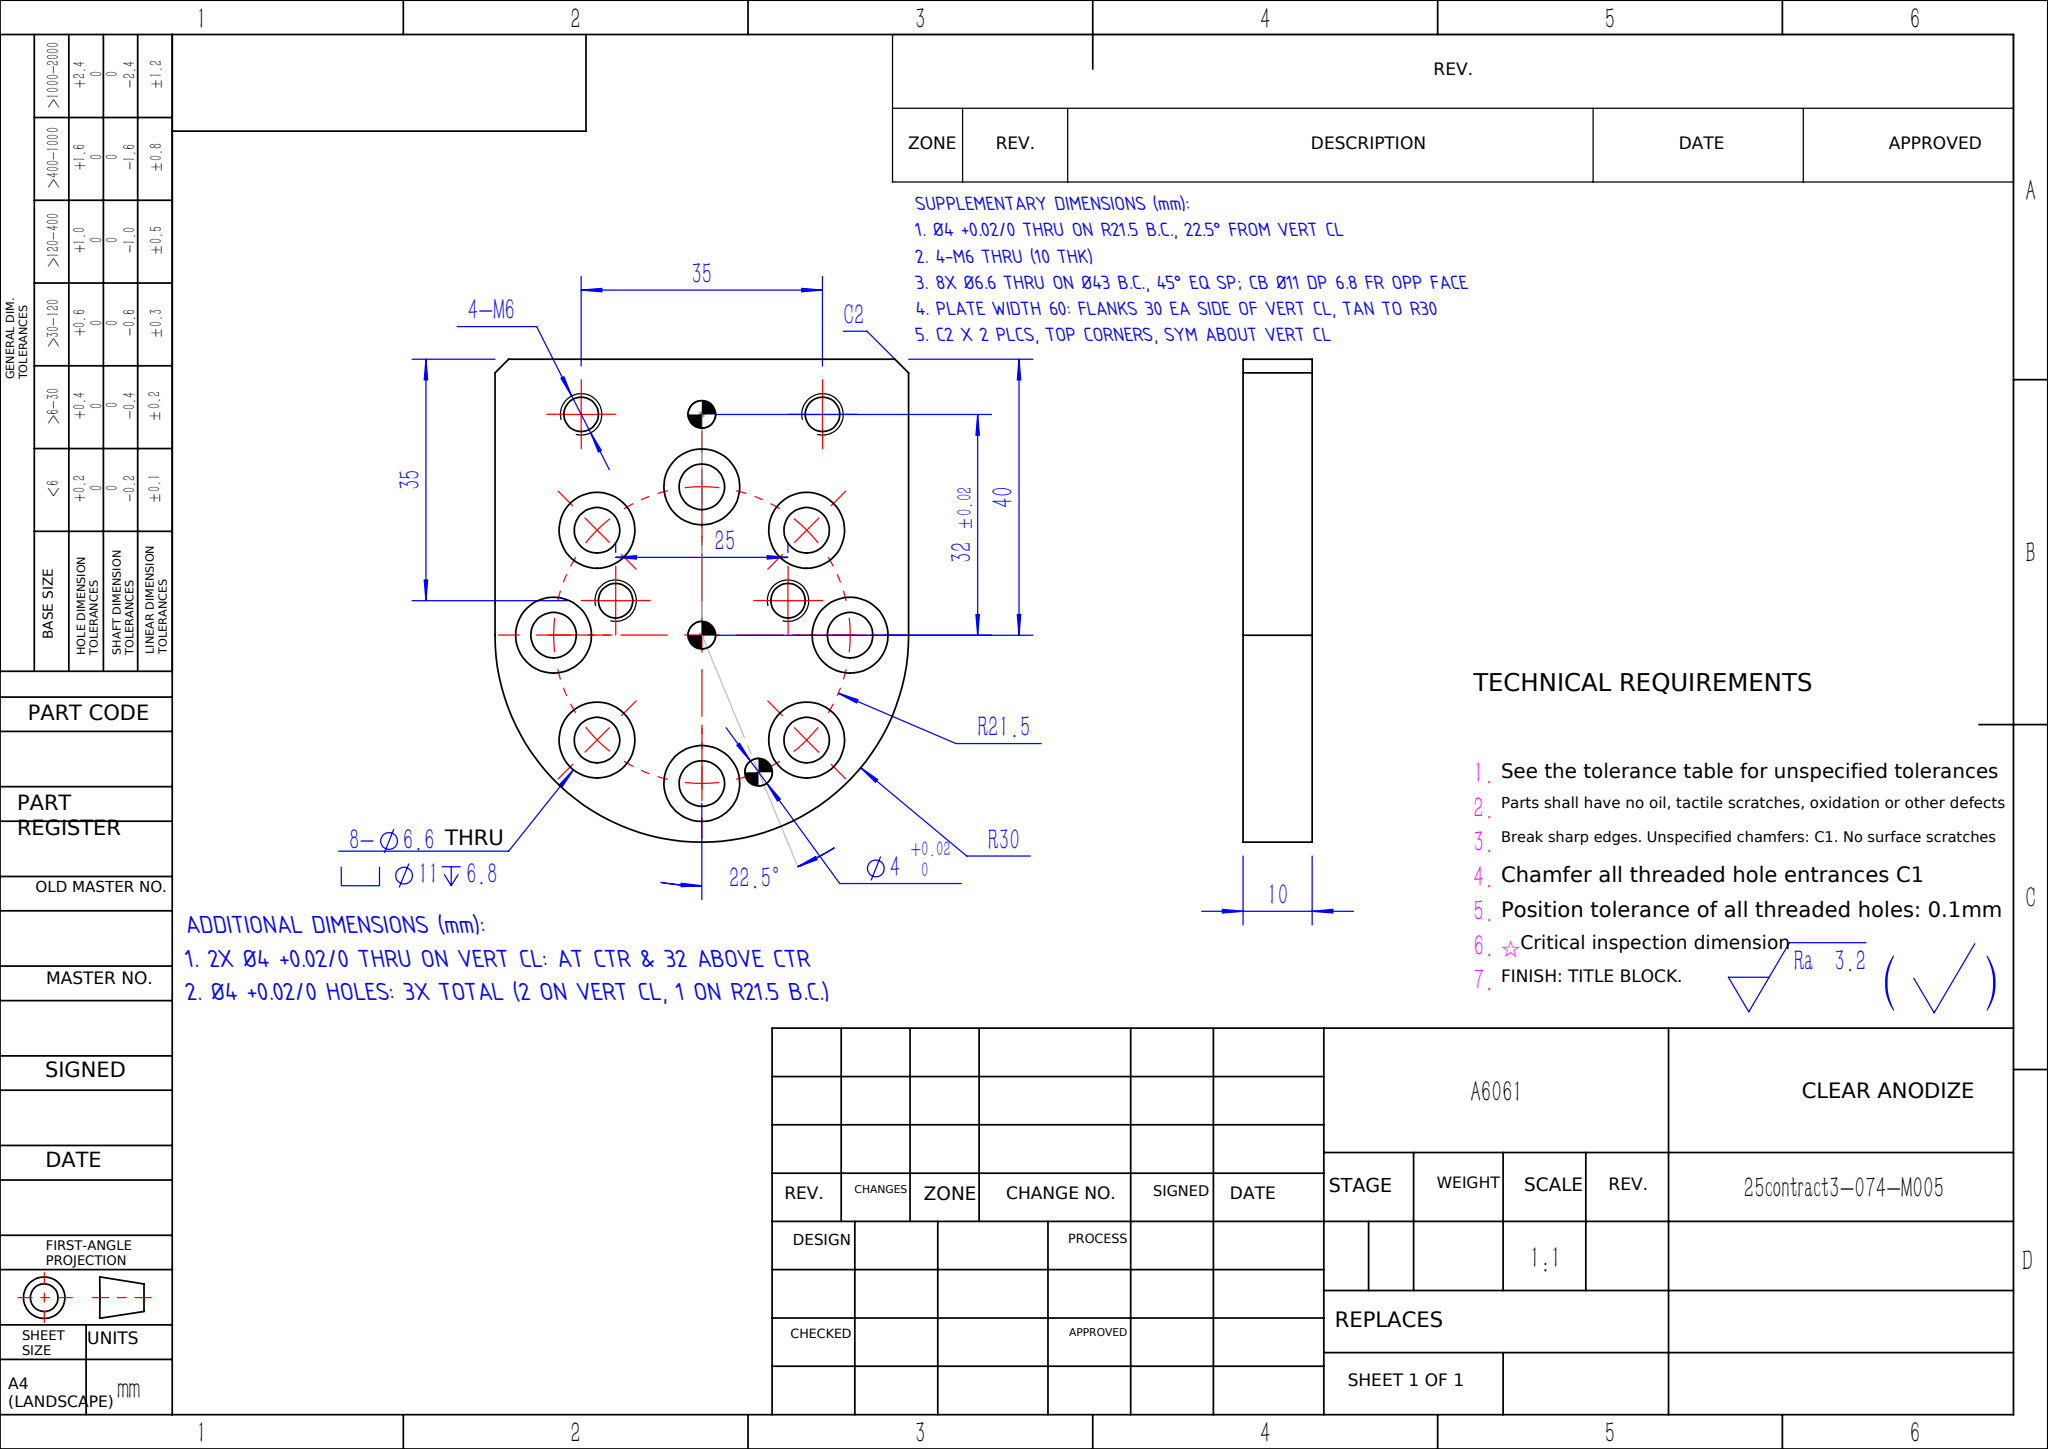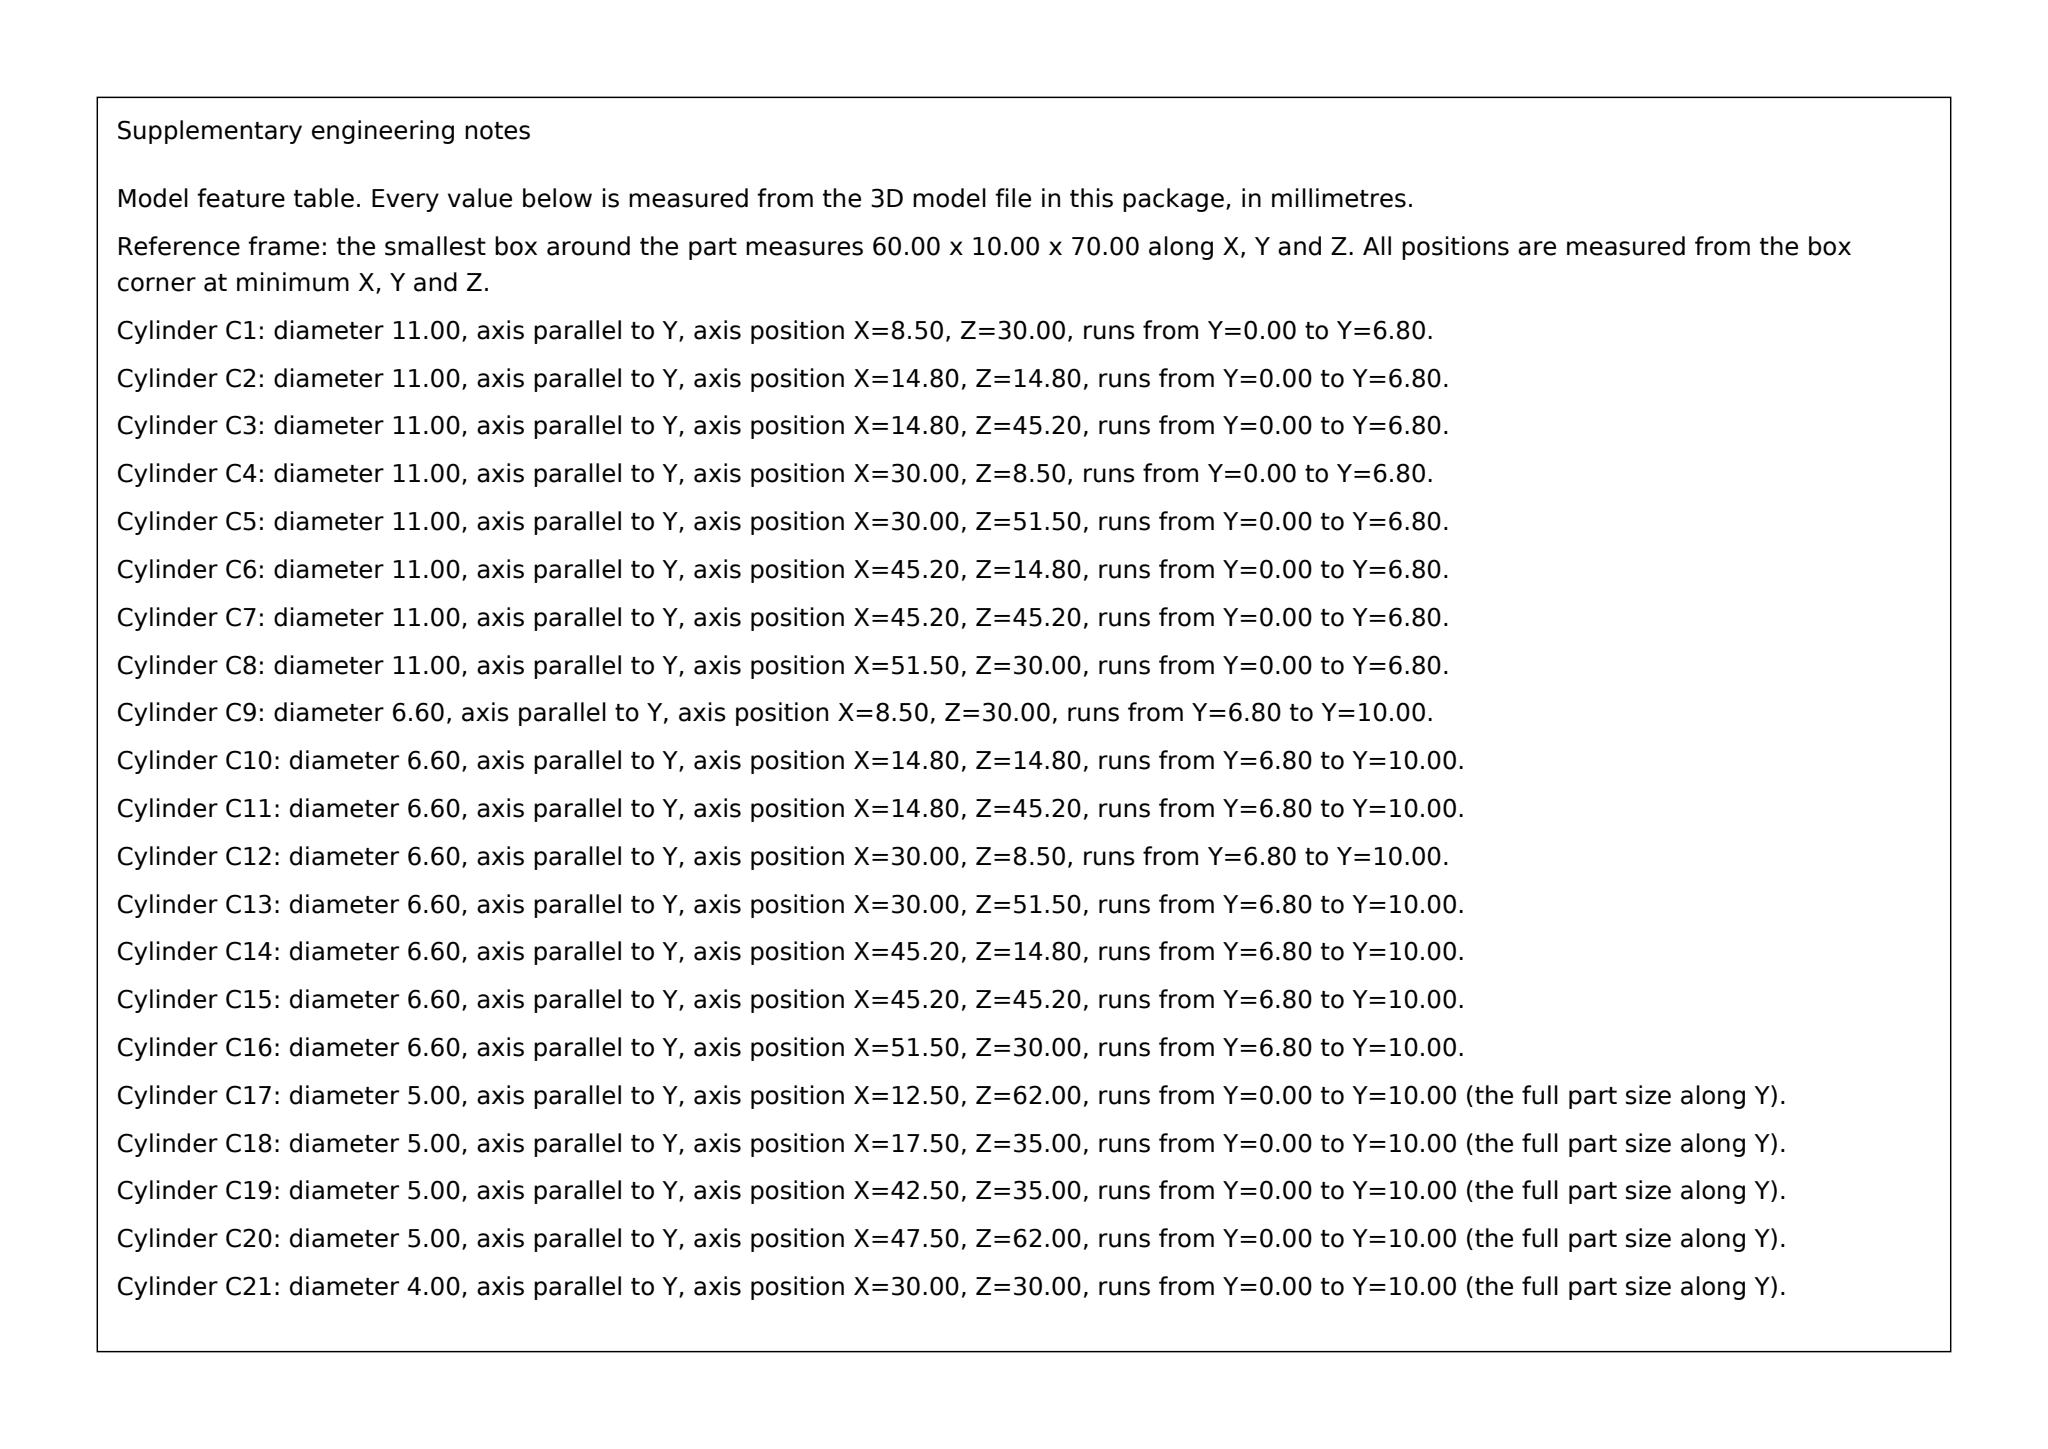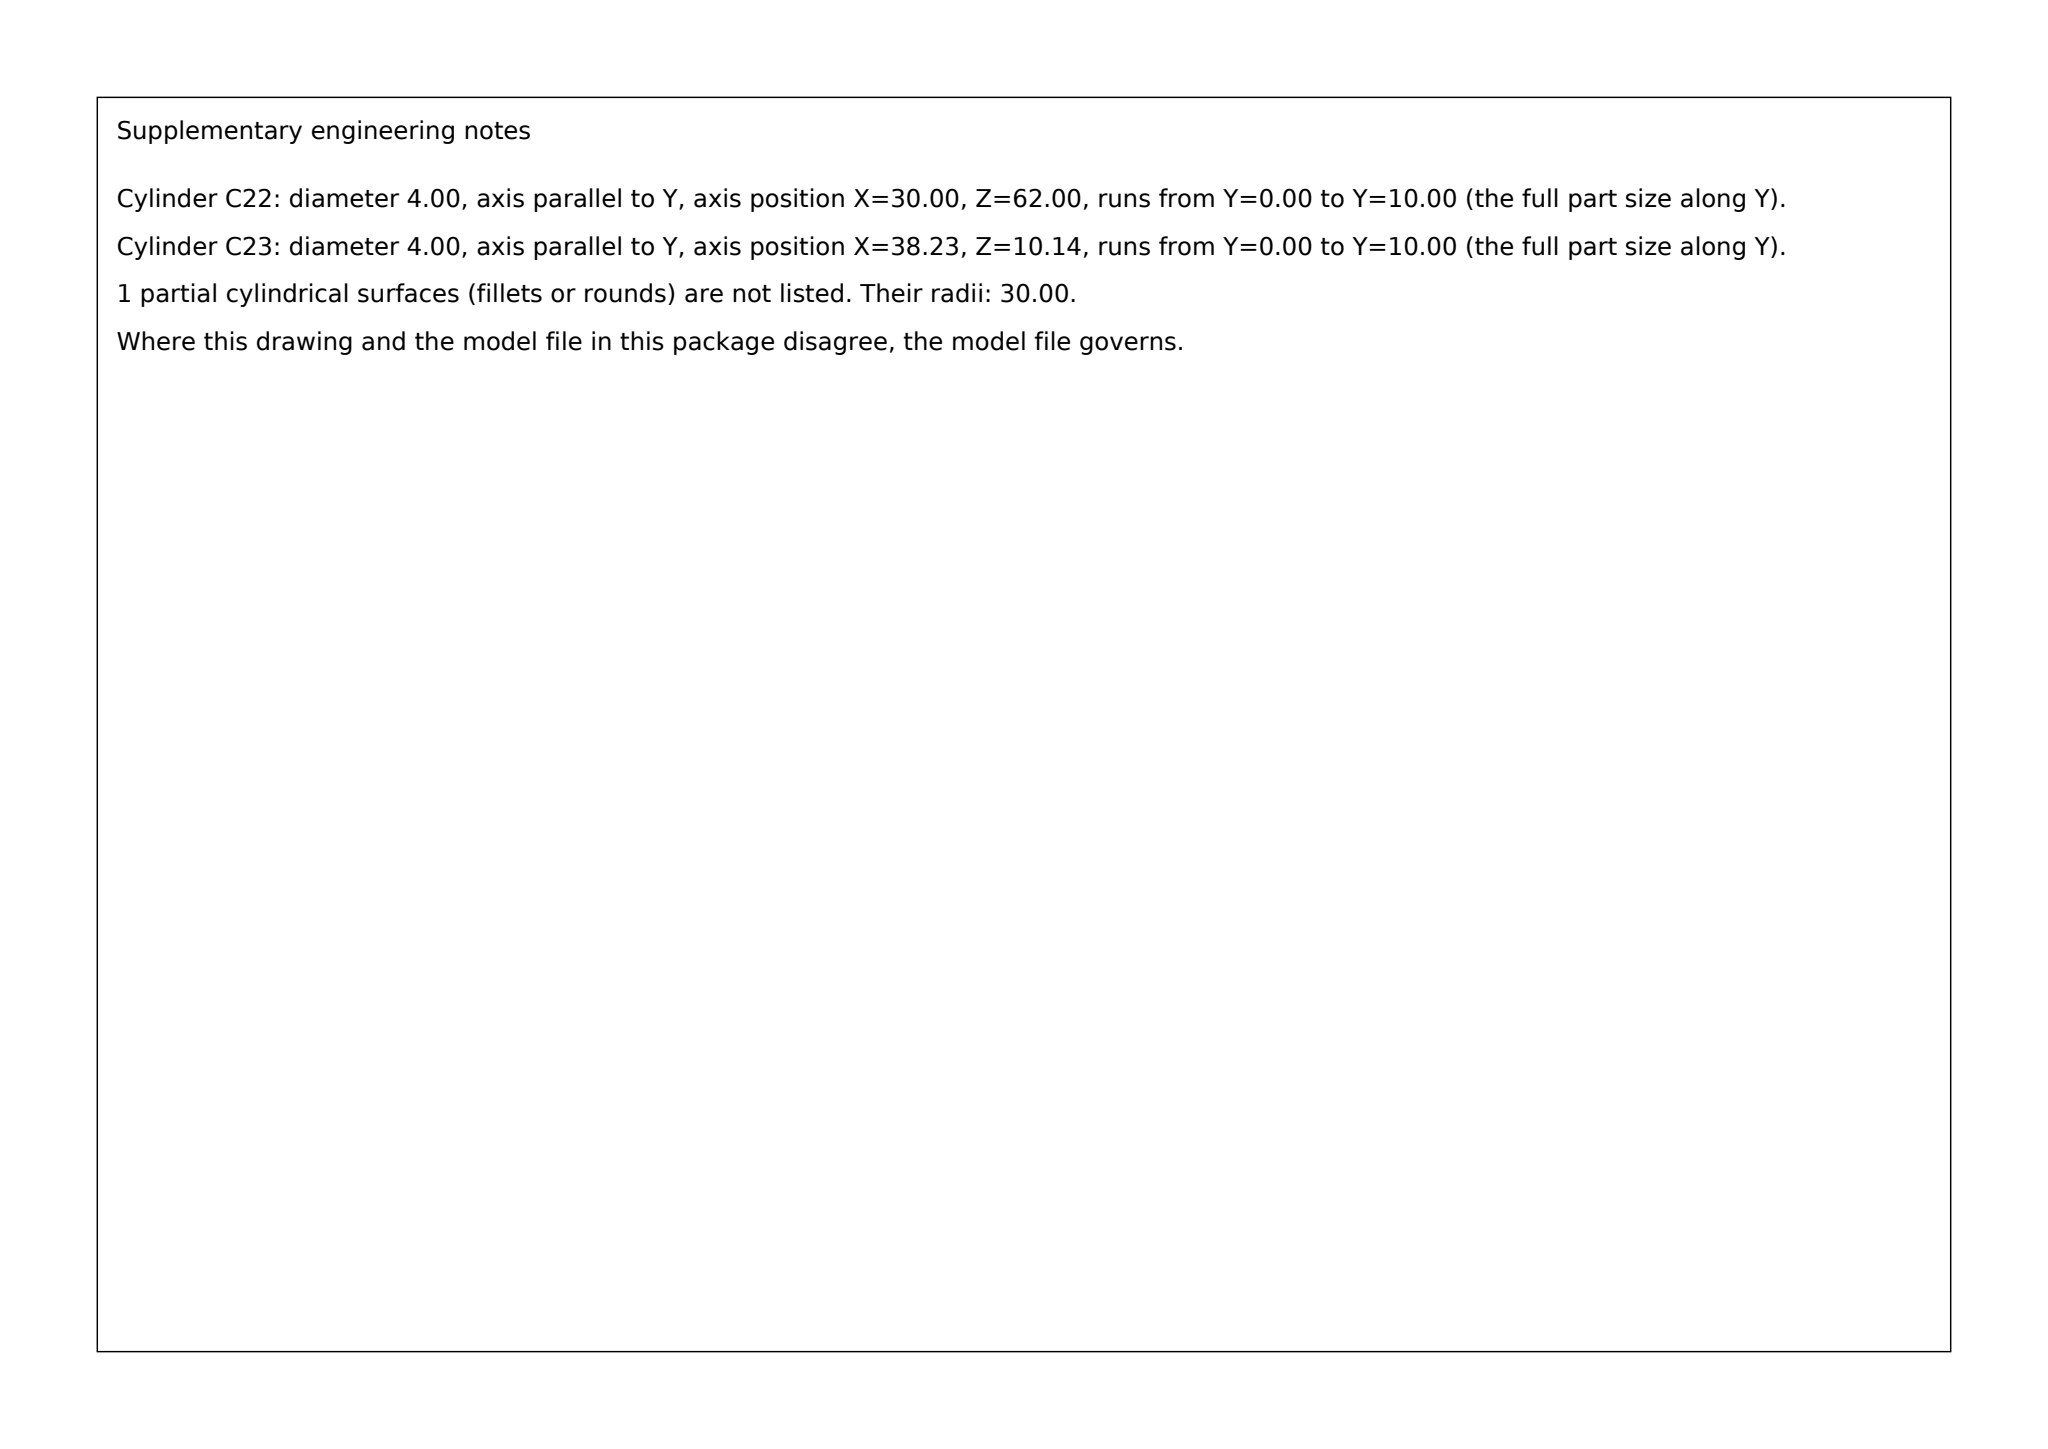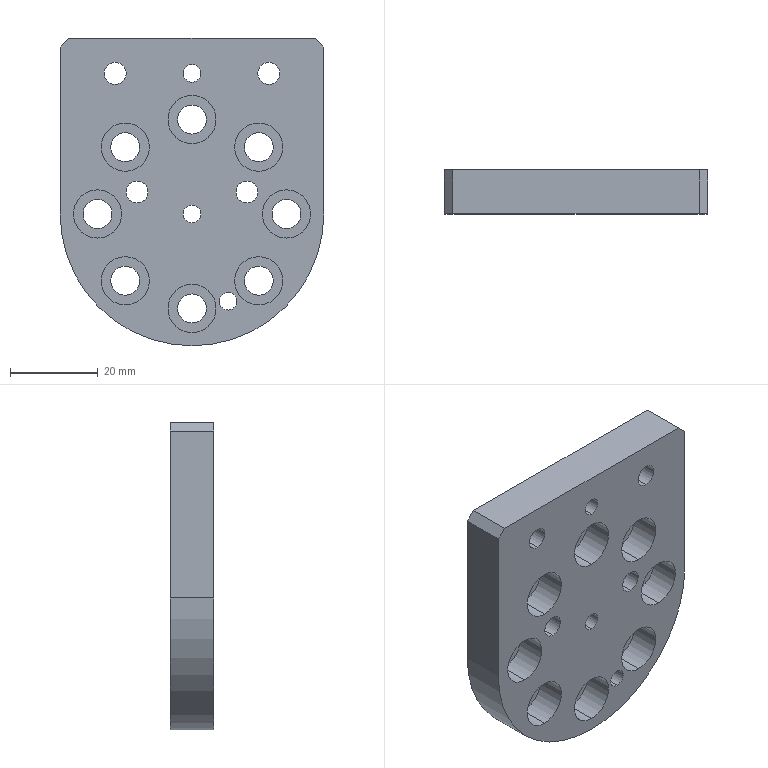Part | SolidWorks | mm | 1 solid | 63 faces | box 60 x 10 x 70 mm | volume 30889 mm3 | cylinder 48 | plane 15 | commonest cylinder face diameters 11 x16 6.6 x16 5 x8 4 x6 60 x2